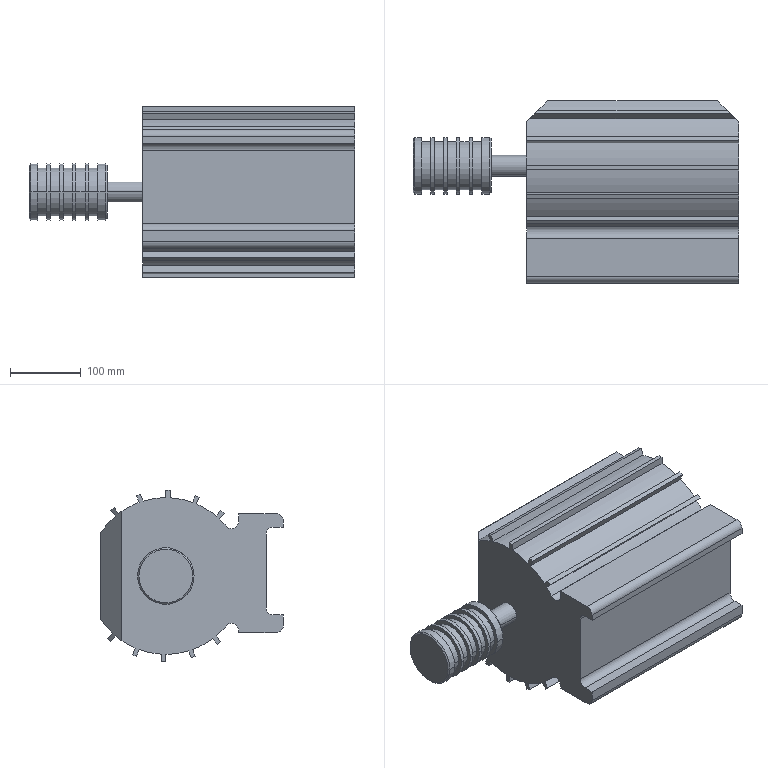Component | SolidWorks | Motor-1 | 1 solid | 102 faces | box 460 x 258 x 242 mm | volume 13903649 mm3 | plane 56 | cylinder 42 | cone 4 | commonest cylinder face diameters 80 x12 221.411 x12 68 x10 20 x6 29.505 x2
build123d program:
from build123d import *

# Parameters (mm, degrees)
BOSS_EXTRUDE1_DEPTH = 300
SKETCH2_W           = 24
SKETCH2_H           = 124
CUT_EXTRUDE1_DEPTH  = 370.995
CHAMFER1_SIZE       = 30
CHAMFER2_SIZE2      = 2
CHAMFER2_SIZE       = 2
FILLET1_R           = 10


with BuildPart() as part:
    # Sketch1 → Boss-Extrude1 (new body)
    with BuildSketch(Plane.XY.offset(-83.732)):
        with BuildLine():
            Line((-112.491, 74.116), (-175.491, 74.116))
            Line((-175.491, 74.116), (-175.491, -93.884))
            Line((-175.491, -93.884), (-112.491, -93.884))
            Line((-112.491, -93.884), (-112.491, -82.83))
            ThreePointArc((-112.491, -82.83), (-105.878, -73.422), (-94.786, -76.456))
            ThreePointArc((-94.786, -76.456), (-90.127, -81.735), (-85.142, -86.708))
            Line((-85.142, -86.708), (-91.864, -94.718))
            Line((-91.864, -94.718), (-87.268, -98.575))
            Line((-87.268, -98.575), (-80.651, -90.689))
            ThreePointArc((-80.651, -90.689), (-67.422, -100.222), (-52.937, -107.708))
            Line((-52.937, -107.708), (-56.513, -117.534))
            Line((-56.513, -117.534), (-50.875, -119.586))
            Line((-50.875, -119.586), (-47.354, -109.913))
            ThreePointArc((-47.354, -109.913), (-31.663, -114.346), (-15.491, -116.426))
            Line((-15.491, -116.426), (-15.491, -126.884))
            Line((-15.491, -126.884), (-9.491, -126.884))
            Line((-9.491, -126.884), (-9.491, -116.589))
            ThreePointArc((-9.491, -116.589), (6.771, -115.388), (22.679, -111.812))
            Line((22.679, -111.812), (26.256, -121.639))
            Line((26.256, -121.639), (31.894, -119.586))
            Line((31.894, -119.586), (28.373, -109.913))
            ThreePointArc((28.373, -109.913), (43.243, -103.223), (56.969, -94.421))
            Line((56.969, -94.421), (63.69, -102.432))
            Line((63.69, -102.432), (68.287, -98.575))
            Line((68.287, -98.575), (61.669, -90.689))
            ThreePointArc((61.669, -90.689), (72.912, -79.813), (82.509, -67.46))
            Line((82.509, -67.46), (82.509, 55.693))
            ThreePointArc((82.509, 55.693), (74.886, 65.784), (66.161, 74.94))
            Line((66.161, 74.94), (72.883, 82.951))
            Line((72.883, 82.951), (68.287, 86.808))
            Line((68.287, 86.808), (61.669, 78.922))
            ThreePointArc((61.669, 78.922), (48.441, 88.454), (33.955, 95.941))
            Line((33.955, 95.941), (37.532, 105.767))
            Line((37.532, 105.767), (31.894, 107.819))
            Line((31.894, 107.819), (28.373, 98.146))
            ThreePointArc((28.373, 98.146), (12.682, 102.579), (-3.491, 104.659))
            Line((-3.491, 104.659), (-3.491, 115.116))
            Line((-3.491, 115.116), (-9.491, 115.116))
            Line((-9.491, 115.116), (-9.491, 104.822))
            ThreePointArc((-9.491, 104.822), (-25.752, 103.621), (-41.66, 100.045))
            Line((-41.66, 100.045), (-45.237, 109.871))
            Line((-45.237, 109.871), (-50.875, 107.819))
            Line((-50.875, 107.819), (-47.354, 98.146))
            ThreePointArc((-47.354, 98.146), (-62.224, 91.455), (-75.95, 82.654))
            Line((-75.95, 82.654), (-82.672, 90.665))
            Line((-82.672, 90.665), (-87.268, 86.808))
            Line((-87.268, 86.808), (-80.651, 78.922))
            ThreePointArc((-80.651, 78.922), (-88.041, 72.126), (-94.786, 64.688))
            ThreePointArc((-94.786, 64.688), (-105.878, 61.655), (-112.491, 71.063))
            Line((-112.491, 71.063), (-112.491, 74.116))
        make_face()
    extrude(amount=-BOSS_EXTRUDE1_DEPTH)

    # Sketch2 → Cut-Extrude1 (cut, through all)
    with BuildSketch(Plane(origin=(0, 0, -383.732), x_dir=(-1, 0, 0), z_dir=(0, 0, -1))):
        with Locations((163.491, -12.884)):
            Rectangle(SKETCH2_W, SKETCH2_H)
    extrude(amount=-CUT_EXTRUDE1_DEPTH, mode=Mode.SUBTRACT)

    # Sketch3 → Revolve1 (revolve)
    with BuildSketch(Plane.XZ.offset(5.884), mode=Mode.PRIVATE) as revolve1_sk:
        Polygon((30.509, 76.268), (-9.491, 76.268), (-9.491, -83.732), (5.262, -83.732), (5.262, -33.732), (30.509, -33.732), (30.509, -20.552), (24.509, -20.552), (24.509, -7.552), (30.509, -7.552), (30.509, -2.552), (24.509, -2.552), (24.509, 10.448), (30.509, 10.448), (30.509, 15.448), (24.509, 15.448), (24.509, 28.448), (30.509, 28.448), (30.509, 33.448), (24.509, 33.448), (24.509, 46.448), (30.509, 46.448), (30.509, 51.448), (24.509, 51.448), (24.509, 64.448), (30.509, 64.448), align=None)
    revolve(revolve1_sk.sketch.rotate(Axis((-9.491, -5.884, 76.268), (0, 0, -1)), 180), axis=Axis((-9.491, -5.884, 76.268), (0, 0, -1)))

    # Chamfer1
    chamfer1_edges = [part.edges().sort_by_distance(p)[0] for p in [
        (82.509, -5.884, -83.732),
        (82.509, -5.884, -383.732),
    ]]
    chamfer(chamfer1_edges, length=CHAMFER1_SIZE)

    # Chamfer2
    chamfer2_edges = [part.edges().sort_by_distance(p)[0] for p in [
        (30.509, -5.884, 76.268),
        (30.509, -5.884, -33.732),
    ]]
    chamfer(chamfer2_edges, length=CHAMFER2_SIZE, length2=CHAMFER2_SIZE2)

    # Fillet1
    fillet1_edges = [part.edges().sort_by_distance(p)[0] for p in [
        (-151.491, -74.884, -233.732),
        (-151.491, 49.116, -233.732),
        (-175.491, -93.884, -233.732),
        (-175.491, 74.116, -233.732),
    ]]
    fillet(fillet1_edges, radius=FILLET1_R)


solid = part.part

# Placed as in the assembly
solid = solid.moved(Location((-827.071, 1749.526, 701.113), (-90, -90, 0)))